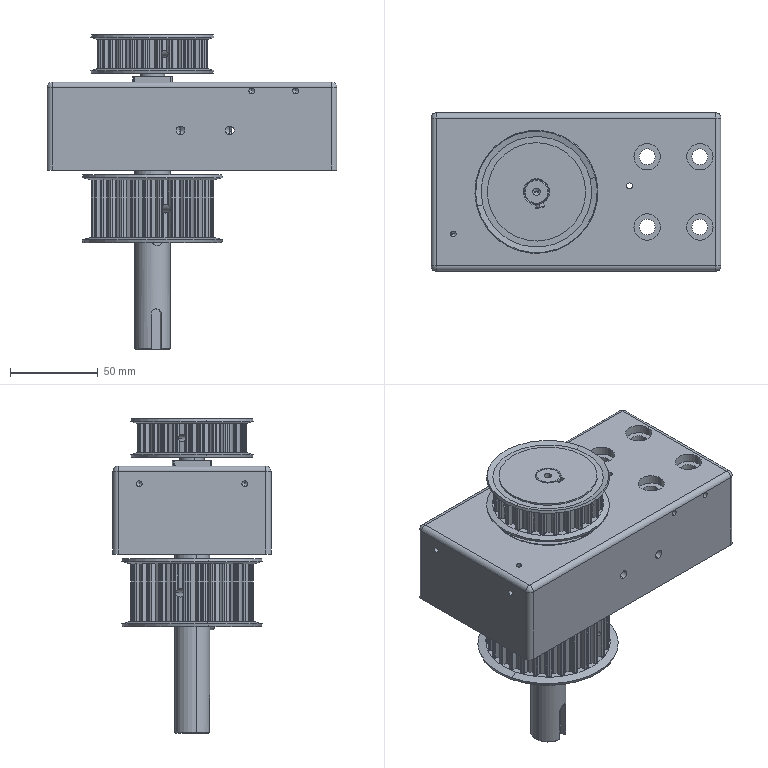Assembly | SolidWorks | mm | 12 component files | 12 solids | 985 faces | box 165 x 90 x 179 mm | volume 737307 mm3 | cylinder 686 | cone 145 | plane 86 | spline 64 | sphere 4 | commonest cylinder face diameters 0.8 x131 1.5 x129 10.6 x111 64.27 x31 5 x29 69.93 x28 56.63 x27 62.29 x25
Bill of materials:
B6-L30 | 1 |  | Slender solid prism with a stadium-shaped (rounded-end) profile and flat parallel faces; looks like a round-ended key.
BAU6003Z | 2 |  | Annular body made of an outer ring and an inner ring that share an axis, with a recessed annular gap between them; looks like a simplified ball bearing.
Carrier1ZDG0406-A03-P83-X1 | 1 | Chrome Plated Rod | Stepped cylindrical shaft with three diameters, keyway slots, and a small hole in the center of the narrow end face.
CarrierB5-L15 | 1 |  | Solid prism with a stadium-shaped (rounded-end) profile and flat parallel faces; shorter and wider than the other key-like part, looks like a round-ended key.
CarrierBKE51-M17 | 1 |  | Square block with chamfered corners and a cylindrical boss underneath, pierced by a large central bore that has a stepped or chamfered entry; a small hole is visible in the bore wall.
CarrierZDG0406-A03-B02-X1 | 1 | 45# | Toothed pulley-like wheel with a flange on each side, a keyed central bore, and one radial hole through the toothed rim.
ZDG0406-A03-B03-X1 | 1 | 45# | Toothed pulley-like wheel with a flange on each side, a keyed central bore, and a radial hole; the toothed face is wider than on unnamed part.
ZDG0406-A03-P06-X1 | 2 | 45# | Flat circular flange with a raised cylindrical hub ring, a large central through bore, and four through holes evenly spaced on a bolt circle.
ZDG0406-A03-P07-X1 | 1 | 45# | Plain cylindrical tube or sleeve with a thin wall and flat end faces.
ZDG0406-A03-P12-X1 | 1 | 45# | Bracket with a U-shaped (channel) section, rounded bend edges, and a perforated top plate: a large central hole surrounded by four small holes, four larger holes, and small holes in the side walls.
Mates:
1. concentric | ZDG0406-A03-P12-X1-1 face at (-22.5, 0, 25) dir (0, 0, -1) r 17.5 | ZDG0406-A03-P06-X1-1 face at (-22.5, 0, -15) dir (0, 0, 1) r 17.5
2. coincident | ZDG0406-A03-P12-X1-1 face at (-22.5, 0, -20) dir (0, 0, -1) | ZDG0406-A03-P06-X1-1 face at (-5, 0, -20) dir (0, 0, 1)
3. coincident | ZDG0406-A03-P06-X1-1 face at (-7, 0, -15) dir (0, 0, 1) | BAU6003Z-1 face at (-22.5, 17.2, -15) dir (0, 0, -1)
4. concentric | ZDG0406-A03-P12-X1-1 face at (-22.5, 0, 25) dir (0, 0, -1) r 17.5 | BAU6003Z-1 face at (-22.5, 0, -5.3) dir (0, 0, -1) r 17.5
5. coincident | ZDG0406-A03-P07-X1-1 face at (-22.5, 0, -5) dir (0, 0, -1) | BAU6003Z-1 face at (-22.5, 8.8, -5) dir (0, 0, 1)
6. concentric | ZDG0406-A03-P12-X1-1 face at (-22.5, 0, 25) dir (0, 0, -1) r 17.5 | ZDG0406-A03-P07-X1-1 face at (-22.5, 0, 5) dir (0, 0, -1) r 10.5
7. coincident | ZDG0406-A03-P07-X1-1 face at (-22.5, 0, 5) dir (0, 0, 1) | BAU6003Z-2 face at (-22.5, 8.8, 5) dir (0, 0, -1)
8. coincident | BAU6003Z-2 face at (-22.5, 10.5, 15) dir (0, 0, 1) | CarrierBKE51-M17-1 face at (-22.5, 0, 15) dir (0, 0, -1)
9. concentric | ZDG0406-A03-P12-X1-1 face at (-22.5, 0, 25) dir (0, 0, -1) r 17.5 | ZDG0406-A03-P06-X1-2 face at (-22.5, 0, 15) dir (0, 0, -1) r 15.5
10. coincident | BAU6003Z-2 face at (-22.5, 17.2, 15) dir (0, 0, 1) | ZDG0406-A03-P06-X1-2 face at (-7, 0, 15) dir (0, 0, -1)
11. coincident | B6-L30-1 face at (-22.449, -12.855, -65) dir (-0.9714, -0.2373, 0) | ZDG0406-A03-B03-X1-1 face at (-23.201, -9.775, -28) dir (0.9714, 0.2373, 0)
12. distance | ZDG0406-A03-B03-X1-1 face at (-22.5, 0, -28) dir (0, 0, 1) | ZDG0406-A03-P12-X1-1 face at (0, 0, -25) dir (0, 0, -1)
13. coincident | CarrierB5-L15-1 face at (-19.122, -3.293, 37) dir (0.9714, 0.2373, 0) | CarrierZDG0406-A03-B02-X1-1 face at (-17.912, -8.247, 52) dir (-0.9714, -0.2373, 0)
14. concentric | ZDG0406-A03-B03-X1-1 face at (-22.5, 0, -66) dir (0, 0, 1) r 10 | Carrier1ZDG0406-A03-P83-X1-1 face at (-22.5, 0, -565.043) dir (0, 0, -1) r 10
15. distance | Carrier1ZDG0406-A03-P83-X1-1 face at (-75.228, 39.106, -127) dir (0, 0, -1) | ZDG0406-A03-B03-X1-1 face at (-15.382, -29.143, -66) dir (0, 0, -1)